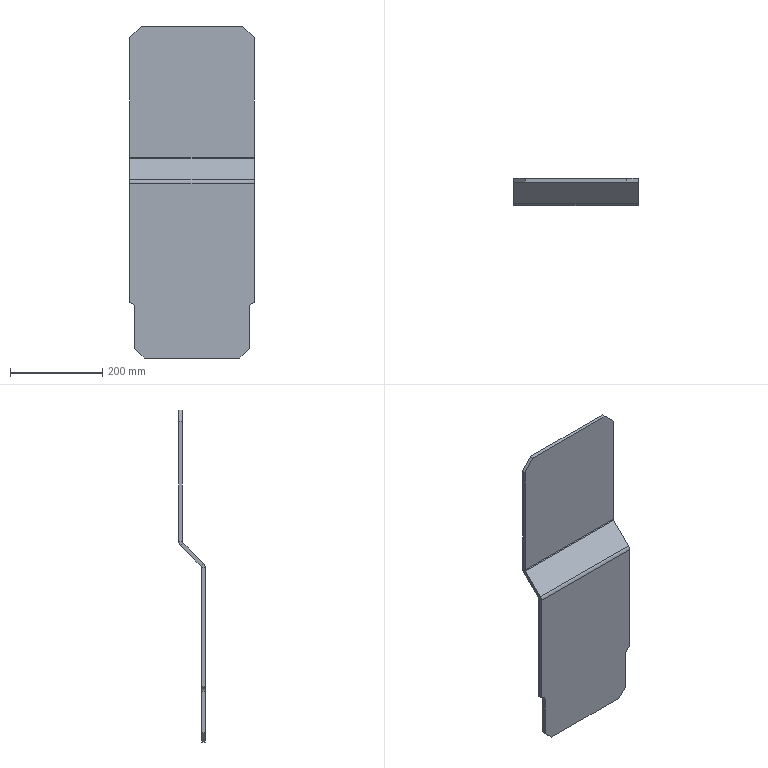Component | SolidWorks | JHK-A1001ConnectingCrossPlate-1 | 1 solid | 30 faces | box 270 x 58 x 720 mm | volume 1569543 mm3 | plane 24 | cylinder 6 | commonest cylinder face diameters 8 x2 24 x2 22 x2 | material Q235A
STEP:
#1=COLOUR_RGB('',0.7922,0.8196,0.9333);
#2=FILL_AREA_STYLE_COLOUR('',#1);
#3=FILL_AREA_STYLE('',(#2));
#4=SURFACE_STYLE_FILL_AREA(#3);
#5=SURFACE_SIDE_STYLE('',(#4));
#6=SURFACE_STYLE_USAGE(.BOTH.,#5);
#7=PRESENTATION_STYLE_ASSIGNMENT((#6));
#8=CARTESIAN_POINT('',(5.315,6.279,2.421));
#9=VERTEX_POINT('',#8);
#10=CARTESIAN_POINT('',(5.315,6.056,2.643));
#11=VERTEX_POINT('',#10);
#12=CARTESIAN_POINT('',(5.315,6.279,2.421));
#13=DIRECTION('',(0.,-0.7071,0.7071));
#14=VECTOR('',#13,39.37);
#15=LINE('',#12,#14);
#16=EDGE_CURVE('',#9,#11,#15,.T.);
#17=ORIENTED_EDGE('',*,*,#16,.F.);
#18=CARTESIAN_POINT('',(5.315,6.417,2.755));
#19=VERTEX_POINT('',#18);
#20=CARTESIAN_POINT('',(5.315,5.945,2.755));
#21=DIRECTION('',(-1.,0.,0.));
#22=DIRECTION('',(0.,0.,-1.));
#23=AXIS2_PLACEMENT_3D('',#20,#21,#22);
#24=CIRCLE('',#23,0.4724);
#25=EDGE_CURVE('',#19,#9,#24,.T.);
#26=ORIENTED_EDGE('',*,*,#25,.F.);
#27=CARTESIAN_POINT('',(5.315,6.102,2.755));
#28=VERTEX_POINT('',#27);
#29=CARTESIAN_POINT('',(5.315,6.102,2.755));
#30=DIRECTION('',(0.,1.,0.));
#31=VECTOR('',#30,39.37);
#32=LINE('',#29,#31);
#33=EDGE_CURVE('',#28,#19,#32,.T.);
#34=ORIENTED_EDGE('',*,*,#33,.F.);
#35=CARTESIAN_POINT('',(5.315,5.945,2.755));
#36=DIRECTION('',(-1.,0.,0.));
#37=DIRECTION('',(0.,0.,-1.));
#38=AXIS2_PLACEMENT_3D('',#35,#36,#37);
#39=CIRCLE('',#38,0.1575);
#40=EDGE_CURVE('',#28,#11,#39,.T.);
#41=ORIENTED_EDGE('',*,*,#40,.T.);
#42=EDGE_LOOP('',(#17,#26,#34,#41));
#43=FACE_OUTER_BOUND('',#42,.T.);
#44=CARTESIAN_POINT('',(5.315,6.279,2.421));
#45=DIRECTION('',(1.,0.,0.));
#46=DIRECTION('',(0.,0.,-1.));
#47=AXIS2_PLACEMENT_3D('',#44,#45,#46);
#48=PLANE('',#47);
#49=ADVANCED_FACE('',(#43),#48,.T.);
#50=CARTESIAN_POINT('',(5.315,4.495,0.6367));
#51=VERTEX_POINT('',#50);
#52=CARTESIAN_POINT('',(5.315,6.417,2.559));
#53=DIRECTION('',(0.,-0.7071,-0.7071));
#54=VECTOR('',#53,39.37);
#55=LINE('',#52,#54);
#56=EDGE_CURVE('',#9,#51,#55,.T.);
#57=ORIENTED_EDGE('',*,*,#56,.F.);
#58=ORIENTED_EDGE('',*,*,#16,.T.);
#59=CARTESIAN_POINT('',(5.315,4.272,0.8594));
#60=VERTEX_POINT('',#59);
#61=CARTESIAN_POINT('',(5.315,6.195,2.782));
#62=DIRECTION('',(0.,-0.7071,-0.7071));
#63=VECTOR('',#62,39.37);
#64=LINE('',#61,#63);
#65=EDGE_CURVE('',#11,#60,#64,.T.);
#66=ORIENTED_EDGE('',*,*,#65,.T.);
#67=CARTESIAN_POINT('',(5.315,4.272,0.8594));
#68=DIRECTION('',(0.,0.7071,-0.7071));
#69=VECTOR('',#68,39.37);
#70=LINE('',#67,#69);
#71=EDGE_CURVE('',#60,#51,#70,.T.);
#72=ORIENTED_EDGE('',*,*,#71,.T.);
#73=EDGE_LOOP('',(#57,#58,#66,#72));
#74=FACE_OUTER_BOUND('',#73,.T.);
#75=CARTESIAN_POINT('',(5.315,6.102,2.755));
#76=DIRECTION('',(1.,0.,0.));
#77=DIRECTION('',(0.,0.,-1.));
#78=AXIS2_PLACEMENT_3D('',#75,#76,#77);
#79=PLANE('',#78);
#80=ADVANCED_FACE('',(#74),#79,.T.);
#81=CARTESIAN_POINT('',(-5.315,6.417,2.755));
#82=VERTEX_POINT('',#81);
#83=CARTESIAN_POINT('',(-5.315,6.102,2.755));
#84=VERTEX_POINT('',#83);
#85=CARTESIAN_POINT('',(-5.315,6.417,2.755));
#86=DIRECTION('',(0.,-1.,-0.));
#87=VECTOR('',#86,39.37);
#88=LINE('',#85,#87);
#89=EDGE_CURVE('',#82,#84,#88,.T.);
#90=ORIENTED_EDGE('',*,*,#89,.F.);
#91=CARTESIAN_POINT('',(-5.315,6.279,2.421));
#92=VERTEX_POINT('',#91);
#93=CARTESIAN_POINT('',(-5.315,5.945,2.755));
#94=DIRECTION('',(-1.,0.,0.));
#95=DIRECTION('',(0.,0.,-1.));
#96=AXIS2_PLACEMENT_3D('',#93,#94,#95);
#97=CIRCLE('',#96,0.4724);
#98=EDGE_CURVE('',#82,#92,#97,.T.);
#99=ORIENTED_EDGE('',*,*,#98,.T.);
#100=CARTESIAN_POINT('',(-5.315,6.056,2.643));
#101=VERTEX_POINT('',#100);
#102=CARTESIAN_POINT('',(-5.315,6.056,2.643));
#103=DIRECTION('',(0.,0.7071,-0.7071));
#104=VECTOR('',#103,39.37);
#105=LINE('',#102,#104);
#106=EDGE_CURVE('',#101,#92,#105,.T.);
#107=ORIENTED_EDGE('',*,*,#106,.F.);
#108=CARTESIAN_POINT('',(-5.315,5.945,2.755));
#109=DIRECTION('',(-1.,0.,0.));
#110=DIRECTION('',(0.,0.,-1.));
#111=AXIS2_PLACEMENT_3D('',#108,#109,#110);
#112=CIRCLE('',#111,0.1575);
#113=EDGE_CURVE('',#84,#101,#112,.T.);
#114=ORIENTED_EDGE('',*,*,#113,.F.);
#115=EDGE_LOOP('',(#90,#99,#107,#114));
#116=FACE_OUTER_BOUND('',#115,.T.);
#117=CARTESIAN_POINT('',(-5.315,6.417,2.755));
#118=DIRECTION('',(-1.,0.,0.));
#119=DIRECTION('',(0.,0.,1.));
#120=AXIS2_PLACEMENT_3D('',#117,#118,#119);
#121=PLANE('',#120);
#122=ADVANCED_FACE('',(#116),#121,.T.);
#123=CARTESIAN_POINT('',(-5.315,6.102,12.992));
#124=VERTEX_POINT('',#123);
#125=CARTESIAN_POINT('',(-5.315,6.102,13.976));
#126=DIRECTION('',(0.,0.,-1.));
#127=VECTOR('',#126,39.37);
#128=LINE('',#125,#127);
#129=EDGE_CURVE('',#124,#84,#128,.T.);
#130=ORIENTED_EDGE('',*,*,#129,.F.);
#131=CARTESIAN_POINT('',(-5.315,6.417,12.992));
#132=VERTEX_POINT('',#131);
#133=CARTESIAN_POINT('',(-5.315,6.056,12.992));
#134=DIRECTION('',(0.,1.,0.));
#135=VECTOR('',#134,39.37);
#136=LINE('',#133,#135);
#137=EDGE_CURVE('',#124,#132,#136,.T.);
#138=ORIENTED_EDGE('',*,*,#137,.T.);
#139=CARTESIAN_POINT('',(-5.315,6.417,13.976));
#140=DIRECTION('',(0.,0.,-1.));
#141=VECTOR('',#140,39.37);
#142=LINE('',#139,#141);
#143=EDGE_CURVE('',#132,#82,#142,.T.);
#144=ORIENTED_EDGE('',*,*,#143,.T.);
#145=ORIENTED_EDGE('',*,*,#89,.T.);
#146=EDGE_LOOP('',(#130,#138,#144,#145));
#147=FACE_OUTER_BOUND('',#146,.T.);
#148=CARTESIAN_POINT('',(-5.315,6.056,2.643));
#149=DIRECTION('',(-1.,0.,0.));
#150=DIRECTION('',(0.,0.,1.));
#151=AXIS2_PLACEMENT_3D('',#148,#149,#150);
#152=PLANE('',#151);
#153=ADVANCED_FACE('',(#147),#152,.T.);
#154=CARTESIAN_POINT('',(5.315,4.449,0.5253));
#155=VERTEX_POINT('',#154);
#156=CARTESIAN_POINT('',(5.315,4.134,0.5253));
#157=VERTEX_POINT('',#156);
#158=CARTESIAN_POINT('',(5.315,4.449,0.5253));
#159=DIRECTION('',(0.,-1.,0.));
#160=VECTOR('',#159,39.37);
#161=LINE('',#158,#160);
#162=EDGE_CURVE('',#155,#157,#161,.T.);
#163=ORIENTED_EDGE('',*,*,#162,.F.);
#164=CARTESIAN_POINT('',(5.315,4.606,0.5253));
#165=DIRECTION('',(1.,0.,0.));
#166=DIRECTION('',(0.,0.,1.));
#167=AXIS2_PLACEMENT_3D('',#164,#165,#166);
#168=CIRCLE('',#167,0.1575);
#169=EDGE_CURVE('',#51,#155,#168,.T.);
#170=ORIENTED_EDGE('',*,*,#169,.F.);
#171=ORIENTED_EDGE('',*,*,#71,.F.);
#172=CARTESIAN_POINT('',(5.315,4.606,0.5253));
#173=DIRECTION('',(1.,0.,0.));
#174=DIRECTION('',(0.,0.,-1.));
#175=AXIS2_PLACEMENT_3D('',#172,#173,#174);
#176=CIRCLE('',#175,0.4724);
#177=EDGE_CURVE('',#60,#157,#176,.T.);
#178=ORIENTED_EDGE('',*,*,#177,.T.);
#179=EDGE_LOOP('',(#163,#170,#171,#178));
#180=FACE_OUTER_BOUND('',#179,.T.);
#181=CARTESIAN_POINT('',(5.315,4.449,0.5253));
#182=DIRECTION('',(1.,0.,0.));
#183=DIRECTION('',(0.,0.,-1.));
#184=AXIS2_PLACEMENT_3D('',#181,#182,#183);
#185=PLANE('',#184);
#186=ADVANCED_FACE('',(#180),#185,.T.);
#187=CARTESIAN_POINT('',(5.315,4.134,-9.646));
#188=VERTEX_POINT('',#187);
#189=CARTESIAN_POINT('',(5.315,4.449,-9.646));
#190=VERTEX_POINT('',#189);
#191=CARTESIAN_POINT('',(5.315,4.134,-9.646));
#192=DIRECTION('',(0.,1.,0.));
#193=VECTOR('',#192,39.37);
#194=LINE('',#191,#193);
#195=EDGE_CURVE('',#188,#190,#194,.T.);
#196=ORIENTED_EDGE('',*,*,#195,.T.);
#197=CARTESIAN_POINT('',(5.315,4.449,0.5906));
#198=DIRECTION('',(0.,0.,-1.));
#199=VECTOR('',#198,39.37);
#200=LINE('',#197,#199);
#201=EDGE_CURVE('',#155,#190,#200,.T.);
#202=ORIENTED_EDGE('',*,*,#201,.F.);
#203=ORIENTED_EDGE('',*,*,#162,.T.);
#204=CARTESIAN_POINT('',(5.315,4.134,0.5906));
#205=DIRECTION('',(0.,0.,-1.));
#206=VECTOR('',#205,39.37);
#207=LINE('',#204,#206);
#208=EDGE_CURVE('',#157,#188,#207,.T.);
#209=ORIENTED_EDGE('',*,*,#208,.T.);
#210=EDGE_LOOP('',(#196,#202,#203,#209));
#211=FACE_OUTER_BOUND('',#210,.T.);
#212=CARTESIAN_POINT('',(5.315,4.272,0.8594));
#213=DIRECTION('',(1.,0.,0.));
#214=DIRECTION('',(0.,0.,-1.));
#215=AXIS2_PLACEMENT_3D('',#212,#213,#214);
#216=PLANE('',#215);
#217=ADVANCED_FACE('',(#211),#216,.T.);
#218=CARTESIAN_POINT('',(-5.315,4.495,0.6367));
#219=VERTEX_POINT('',#218);
#220=CARTESIAN_POINT('',(-5.315,4.272,0.8594));
#221=VERTEX_POINT('',#220);
#222=CARTESIAN_POINT('',(-5.315,4.495,0.6367));
#223=DIRECTION('',(0.,-0.7071,0.7071));
#224=VECTOR('',#223,39.37);
#225=LINE('',#222,#224);
#226=EDGE_CURVE('',#219,#221,#225,.T.);
#227=ORIENTED_EDGE('',*,*,#226,.F.);
#228=CARTESIAN_POINT('',(-5.315,4.449,0.5253));
#229=VERTEX_POINT('',#228);
#230=CARTESIAN_POINT('',(-5.315,4.606,0.5253));
#231=DIRECTION('',(1.,0.,0.));
#232=DIRECTION('',(0.,0.,1.));
#233=AXIS2_PLACEMENT_3D('',#230,#231,#232);
#234=CIRCLE('',#233,0.1575);
#235=EDGE_CURVE('',#219,#229,#234,.T.);
#236=ORIENTED_EDGE('',*,*,#235,.T.);
#237=CARTESIAN_POINT('',(-5.315,4.134,0.5253));
#238=VERTEX_POINT('',#237);
#239=CARTESIAN_POINT('',(-5.315,4.134,0.5253));
#240=DIRECTION('',(0.,1.,0.));
#241=VECTOR('',#240,39.37);
#242=LINE('',#239,#241);
#243=EDGE_CURVE('',#238,#229,#242,.T.);
#244=ORIENTED_EDGE('',*,*,#243,.F.);
#245=CARTESIAN_POINT('',(-5.315,4.606,0.5253));
#246=DIRECTION('',(1.,0.,0.));
#247=DIRECTION('',(0.,0.,-1.));
#248=AXIS2_PLACEMENT_3D('',#245,#246,#247);
#249=CIRCLE('',#248,0.4724);
#250=EDGE_CURVE('',#221,#238,#249,.T.);
#251=ORIENTED_EDGE('',*,*,#250,.F.);
#252=EDGE_LOOP('',(#227,#236,#244,#251));
#253=FACE_OUTER_BOUND('',#252,.T.);
#254=CARTESIAN_POINT('',(-5.315,4.495,0.6367));
#255=DIRECTION('',(-1.,0.,0.));
#256=DIRECTION('',(0.,0.,1.));
#257=AXIS2_PLACEMENT_3D('',#254,#255,#256);
#258=PLANE('',#257);
#259=ADVANCED_FACE('',(#253),#258,.T.);
#260=CARTESIAN_POINT('',(-5.315,6.417,2.559));
#261=DIRECTION('',(0.,-0.7071,-0.7071));
#262=VECTOR('',#261,39.37);
#263=LINE('',#260,#262);
#264=EDGE_CURVE('',#92,#219,#263,.T.);
#265=ORIENTED_EDGE('',*,*,#264,.T.);
#266=ORIENTED_EDGE('',*,*,#226,.T.);
#267=CARTESIAN_POINT('',(-5.315,6.195,2.782));
#268=DIRECTION('',(0.,-0.7071,-0.7071));
#269=VECTOR('',#268,39.37);
#270=LINE('',#267,#269);
#271=EDGE_CURVE('',#101,#221,#270,.T.);
#272=ORIENTED_EDGE('',*,*,#271,.F.);
#273=ORIENTED_EDGE('',*,*,#106,.T.);
#274=EDGE_LOOP('',(#265,#266,#272,#273));
#275=FACE_OUTER_BOUND('',#274,.T.);
#276=CARTESIAN_POINT('',(-5.315,4.134,0.5253));
#277=DIRECTION('',(-1.,0.,0.));
#278=DIRECTION('',(0.,0.,1.));
#279=AXIS2_PLACEMENT_3D('',#276,#277,#278);
#280=PLANE('',#279);
#281=ADVANCED_FACE('',(#275),#280,.T.);
#282=CARTESIAN_POINT('',(-4.882,4.134,-10.079));
#283=VERTEX_POINT('',#282);
#284=CARTESIAN_POINT('',(-4.882,4.134,-13.583));
#285=VERTEX_POINT('',#284);
#286=CARTESIAN_POINT('',(-4.882,4.134,-14.37));
#287=DIRECTION('',(-0.,0.,-1.));
#288=VECTOR('',#287,39.37);
#289=LINE('',#286,#288);
#290=EDGE_CURVE('',#283,#285,#289,.T.);
#291=ORIENTED_EDGE('',*,*,#290,.T.);
#292=CARTESIAN_POINT('',(-4.094,4.134,-14.37));
#293=VERTEX_POINT('',#292);
#294=CARTESIAN_POINT('',(-4.094,4.134,-14.37));
#295=DIRECTION('',(0.7071,0.,-0.7071));
#296=VECTOR('',#295,39.37);
#297=LINE('',#294,#296);
#298=EDGE_CURVE('',#285,#293,#297,.T.);
#299=ORIENTED_EDGE('',*,*,#298,.T.);
#300=CARTESIAN_POINT('',(4.094,4.134,-14.37));
#301=VERTEX_POINT('',#300);
#302=CARTESIAN_POINT('',(5.315,4.134,-14.37));
#303=DIRECTION('',(-1.,0.,0.));
#304=VECTOR('',#303,39.37);
#305=LINE('',#302,#304);
#306=EDGE_CURVE('',#301,#293,#305,.T.);
#307=ORIENTED_EDGE('',*,*,#306,.F.);
#308=CARTESIAN_POINT('',(4.882,4.134,-13.583));
#309=VERTEX_POINT('',#308);
#310=CARTESIAN_POINT('',(4.882,4.134,-13.583));
#311=DIRECTION('',(0.7071,-0.,0.7071));
#312=VECTOR('',#311,39.37);
#313=LINE('',#310,#312);
#314=EDGE_CURVE('',#301,#309,#313,.T.);
#315=ORIENTED_EDGE('',*,*,#314,.T.);
#316=CARTESIAN_POINT('',(4.882,4.134,-10.079));
#317=VERTEX_POINT('',#316);
#318=CARTESIAN_POINT('',(4.882,4.134,-14.37));
#319=DIRECTION('',(0.,0.,1.));
#320=VECTOR('',#319,39.37);
#321=LINE('',#318,#320);
#322=EDGE_CURVE('',#309,#317,#321,.T.);
#323=ORIENTED_EDGE('',*,*,#322,.T.);
#324=CARTESIAN_POINT('',(5.315,4.134,-10.079));
#325=DIRECTION('',(0.,1.,0.));
#326=DIRECTION('',(0.,0.,1.));
#327=AXIS2_PLACEMENT_3D('',#324,#325,#326);
#328=CIRCLE('',#327,0.4331);
#329=EDGE_CURVE('',#317,#188,#328,.T.);
#330=ORIENTED_EDGE('',*,*,#329,.T.);
#331=ORIENTED_EDGE('',*,*,#208,.F.);
#332=CARTESIAN_POINT('',(5.315,4.134,0.5253));
#333=DIRECTION('',(-1.,0.,0.));
#334=VECTOR('',#333,39.37);
#335=LINE('',#332,#334);
#336=EDGE_CURVE('',#157,#238,#335,.T.);
#337=ORIENTED_EDGE('',*,*,#336,.T.);
#338=CARTESIAN_POINT('',(-5.315,4.134,-9.646));
#339=VERTEX_POINT('',#338);
#340=CARTESIAN_POINT('',(-5.315,4.134,0.5906));
#341=DIRECTION('',(0.,0.,-1.));
#342=VECTOR('',#341,39.37);
#343=LINE('',#340,#342);
#344=EDGE_CURVE('',#238,#339,#343,.T.);
#345=ORIENTED_EDGE('',*,*,#344,.T.);
#346=CARTESIAN_POINT('',(-5.315,4.134,-10.079));
#347=DIRECTION('',(0.,1.,0.));
#348=DIRECTION('',(0.,0.,1.));
#349=AXIS2_PLACEMENT_3D('',#346,#347,#348);
#350=CIRCLE('',#349,0.4331);
#351=EDGE_CURVE('',#339,#283,#350,.T.);
#352=ORIENTED_EDGE('',*,*,#351,.T.);
#353=EDGE_LOOP('',(#291,#299,#307,#315,#323,#330,#331,#337,#345,#352));
#354=FACE_OUTER_BOUND('',#353,.T.);
#355=CARTESIAN_POINT('',(5.315,4.134,0.5906));
#356=DIRECTION('',(0.,1.,0.));
#357=DIRECTION('',(0.,-0.,1.));
#358=AXIS2_PLACEMENT_3D('',#355,#356,#357);
#359=PLANE('',#358);
#360=ADVANCED_FACE('',(#354),#359,.F.);
#361=ORIENTED_EDGE('',*,*,#306,.T.);
#362=CARTESIAN_POINT('',(-4.094,4.449,-14.37));
#363=VERTEX_POINT('',#362);
#364=CARTESIAN_POINT('',(-4.094,4.449,-14.37));
#365=DIRECTION('',(0.,1.,0.));
#366=VECTOR('',#365,39.37);
#367=LINE('',#364,#366);
#368=EDGE_CURVE('',#293,#363,#367,.T.);
#369=ORIENTED_EDGE('',*,*,#368,.T.);
#370=CARTESIAN_POINT('',(4.094,4.449,-14.37));
#371=VERTEX_POINT('',#370);
#372=CARTESIAN_POINT('',(5.315,4.449,-14.37));
#373=DIRECTION('',(-1.,0.,0.));
#374=VECTOR('',#373,39.37);
#375=LINE('',#372,#374);
#376=EDGE_CURVE('',#371,#363,#375,.T.);
#377=ORIENTED_EDGE('',*,*,#376,.F.);
#378=CARTESIAN_POINT('',(4.094,4.134,-14.37));
#379=DIRECTION('',(0.,-1.,0.));
#380=VECTOR('',#379,39.37);
#381=LINE('',#378,#380);
#382=EDGE_CURVE('',#371,#301,#381,.T.);
#383=ORIENTED_EDGE('',*,*,#382,.T.);
#384=EDGE_LOOP('',(#361,#369,#377,#383));
#385=FACE_OUTER_BOUND('',#384,.T.);
#386=CARTESIAN_POINT('',(5.315,4.449,-14.37));
#387=DIRECTION('',(0.,0.,-1.));
#388=DIRECTION('',(-1.,0.,0.));
#389=AXIS2_PLACEMENT_3D('',#386,#387,#388);
#390=PLANE('',#389);
#391=ADVANCED_FACE('',(#385),#390,.T.);
#392=ORIENTED_EDGE('',*,*,#376,.T.);
#393=CARTESIAN_POINT('',(-4.882,4.449,-13.583));
#394=VERTEX_POINT('',#393);
#395=CARTESIAN_POINT('',(-6.87,4.449,-11.594));
#396=DIRECTION('',(-0.7071,-0.,0.7071));
#397=VECTOR('',#396,39.37);
#398=LINE('',#395,#397);
#399=EDGE_CURVE('',#363,#394,#398,.T.);
#400=ORIENTED_EDGE('',*,*,#399,.T.);
#401=CARTESIAN_POINT('',(-4.882,4.449,-10.079));
#402=VERTEX_POINT('',#401);
#403=CARTESIAN_POINT('',(-4.882,4.449,-14.37));
#404=DIRECTION('',(-0.,0.,-1.));
#405=VECTOR('',#404,39.37);
#406=LINE('',#403,#405);
#407=EDGE_CURVE('',#402,#394,#406,.T.);
#408=ORIENTED_EDGE('',*,*,#407,.F.);
#409=CARTESIAN_POINT('',(-5.315,4.449,-9.646));
#410=VERTEX_POINT('',#409);
#411=CARTESIAN_POINT('',(-5.315,4.449,-10.079));
#412=DIRECTION('',(0.,-1.,-0.));
#413=DIRECTION('',(0.,0.,1.));
#414=AXIS2_PLACEMENT_3D('',#411,#412,#413);
#415=CIRCLE('',#414,0.4331);
#416=EDGE_CURVE('',#402,#410,#415,.T.);
#417=ORIENTED_EDGE('',*,*,#416,.T.);
#418=CARTESIAN_POINT('',(-5.315,4.449,0.5906));
#419=DIRECTION('',(0.,0.,-1.));
#420=VECTOR('',#419,39.37);
#421=LINE('',#418,#420);
#422=EDGE_CURVE('',#229,#410,#421,.T.);
#423=ORIENTED_EDGE('',*,*,#422,.F.);
#424=CARTESIAN_POINT('',(5.315,4.449,0.5253));
#425=DIRECTION('',(-1.,0.,0.));
#426=VECTOR('',#425,39.37);
#427=LINE('',#424,#426);
#428=EDGE_CURVE('',#155,#229,#427,.T.);
#429=ORIENTED_EDGE('',*,*,#428,.F.);
#430=ORIENTED_EDGE('',*,*,#201,.T.);
#431=CARTESIAN_POINT('',(4.882,4.449,-10.079));
#432=VERTEX_POINT('',#431);
#433=CARTESIAN_POINT('',(5.315,4.449,-10.079));
#434=DIRECTION('',(0.,-1.,-0.));
#435=DIRECTION('',(0.,0.,1.));
#436=AXIS2_PLACEMENT_3D('',#433,#434,#435);
#437=CIRCLE('',#436,0.4331);
#438=EDGE_CURVE('',#190,#432,#437,.T.);
#439=ORIENTED_EDGE('',*,*,#438,.T.);
#440=CARTESIAN_POINT('',(4.882,4.449,-13.583));
#441=VERTEX_POINT('',#440);
#442=CARTESIAN_POINT('',(4.882,4.449,-14.37));
#443=DIRECTION('',(0.,0.,1.));
#444=VECTOR('',#443,39.37);
#445=LINE('',#442,#444);
#446=EDGE_CURVE('',#441,#432,#445,.T.);
#447=ORIENTED_EDGE('',*,*,#446,.F.);
#448=CARTESIAN_POINT('',(12.185,4.449,-6.28));
#449=DIRECTION('',(-0.7071,0.,-0.7071));
#450=VECTOR('',#449,39.37);
#451=LINE('',#448,#450);
#452=EDGE_CURVE('',#441,#371,#451,.T.);
#453=ORIENTED_EDGE('',*,*,#452,.T.);
#454=EDGE_LOOP('',(#392,#400,#408,#417,#423,#429,#430,#439,#447,#453));
#455=FACE_OUTER_BOUND('',#454,.T.);
#456=CARTESIAN_POINT('',(5.315,4.449,0.5906));
#457=DIRECTION('',(0.,1.,0.));
#458=DIRECTION('',(0.,-0.,1.));
#459=AXIS2_PLACEMENT_3D('',#456,#457,#458);
#460=PLANE('',#459);
#461=ADVANCED_FACE('',(#455),#460,.T.);
#462=ORIENTED_EDGE('',*,*,#235,.F.);
#463=CARTESIAN_POINT('',(5.315,4.495,0.6367));
#464=DIRECTION('',(-1.,0.,0.));
#465=VECTOR('',#464,39.37);
#466=LINE('',#463,#465);
#467=EDGE_CURVE('',#51,#219,#466,.T.);
#468=ORIENTED_EDGE('',*,*,#467,.F.);
#469=ORIENTED_EDGE('',*,*,#169,.T.);
#470=ORIENTED_EDGE('',*,*,#428,.T.);
#471=EDGE_LOOP('',(#462,#468,#469,#470));
#472=FACE_OUTER_BOUND('',#471,.T.);
#473=CARTESIAN_POINT('',(5.315,4.606,0.5253));
#474=DIRECTION('',(-1.,0.,0.));
#475=DIRECTION('',(0.,0.,1.));
#476=AXIS2_PLACEMENT_3D('',#473,#474,#475);
#477=CYLINDRICAL_SURFACE('',#476,0.1575);
#478=ADVANCED_FACE('',(#472),#477,.F.);
#479=ORIENTED_EDGE('',*,*,#264,.F.);
#480=CARTESIAN_POINT('',(5.315,6.279,2.421));
#481=DIRECTION('',(-1.,0.,0.));
#482=VECTOR('',#481,39.37);
#483=LINE('',#480,#482);
#484=EDGE_CURVE('',#9,#92,#483,.T.);
#485=ORIENTED_EDGE('',*,*,#484,.F.);
#486=ORIENTED_EDGE('',*,*,#56,.T.);
#487=ORIENTED_EDGE('',*,*,#467,.T.);
#488=EDGE_LOOP('',(#479,#485,#486,#487));
#489=FACE_OUTER_BOUND('',#488,.T.);
#490=CARTESIAN_POINT('',(5.315,6.417,2.559));
#491=DIRECTION('',(0.,0.7071,-0.7071));
#492=DIRECTION('',(0.,0.7071,0.7071));
#493=AXIS2_PLACEMENT_3D('',#490,#491,#492);
#494=PLANE('',#493);
#495=ADVANCED_FACE('',(#489),#494,.T.);
#496=ORIENTED_EDGE('',*,*,#98,.F.);
#497=CARTESIAN_POINT('',(5.315,6.417,2.755));
#498=DIRECTION('',(-1.,0.,0.));
#499=VECTOR('',#498,39.37);
#500=LINE('',#497,#499);
#501=EDGE_CURVE('',#19,#82,#500,.T.);
#502=ORIENTED_EDGE('',*,*,#501,.F.);
#503=ORIENTED_EDGE('',*,*,#25,.T.);
#504=ORIENTED_EDGE('',*,*,#484,.T.);
#505=EDGE_LOOP('',(#496,#502,#503,#504));
#506=FACE_OUTER_BOUND('',#505,.T.);
#507=CARTESIAN_POINT('',(5.315,5.945,2.755));
#508=DIRECTION('',(-1.,0.,0.));
#509=DIRECTION('',(0.,0.,1.));
#510=AXIS2_PLACEMENT_3D('',#507,#508,#509);
#511=CYLINDRICAL_SURFACE('',#510,0.4724);
#512=ADVANCED_FACE('',(#506),#511,.T.);
#513=ORIENTED_EDGE('',*,*,#143,.F.);
#514=CARTESIAN_POINT('',(-4.331,6.417,13.976));
#515=VERTEX_POINT('',#514);
#516=CARTESIAN_POINT('',(0.4921,6.417,18.799));
#517=DIRECTION('',(0.7071,0.,0.7071));
#518=VECTOR('',#517,39.37);
#519=LINE('',#516,#518);
#520=EDGE_CURVE('',#132,#515,#519,.T.);
#521=ORIENTED_EDGE('',*,*,#520,.T.);
#522=CARTESIAN_POINT('',(4.331,6.417,13.976));
#523=VERTEX_POINT('',#522);
#524=CARTESIAN_POINT('',(5.315,6.417,13.976));
#525=DIRECTION('',(-1.,0.,0.));
#526=VECTOR('',#525,39.37);
#527=LINE('',#524,#526);
#528=EDGE_CURVE('',#523,#515,#527,.T.);
#529=ORIENTED_EDGE('',*,*,#528,.F.);
#530=CARTESIAN_POINT('',(5.315,6.417,12.992));
#531=VERTEX_POINT('',#530);
#532=CARTESIAN_POINT('',(4.823,6.417,13.484));
#533=DIRECTION('',(0.7071,0.,-0.7071));
#534=VECTOR('',#533,39.37);
#535=LINE('',#532,#534);
#536=EDGE_CURVE('',#523,#531,#535,.T.);
#537=ORIENTED_EDGE('',*,*,#536,.T.);
#538=CARTESIAN_POINT('',(5.315,6.417,13.976));
#539=DIRECTION('',(0.,0.,-1.));
#540=VECTOR('',#539,39.37);
#541=LINE('',#538,#540);
#542=EDGE_CURVE('',#531,#19,#541,.T.);
#543=ORIENTED_EDGE('',*,*,#542,.T.);
#544=ORIENTED_EDGE('',*,*,#501,.T.);
#545=EDGE_LOOP('',(#513,#521,#529,#537,#543,#544));
#546=FACE_OUTER_BOUND('',#545,.T.);
#547=CARTESIAN_POINT('',(5.315,6.417,13.976));
#548=DIRECTION('',(0.,1.,0.));
#549=DIRECTION('',(0.,0.,1.));
#550=AXIS2_PLACEMENT_3D('',#547,#548,#549);
#551=PLANE('',#550);
#552=ADVANCED_FACE('',(#546),#551,.T.);
#553=ORIENTED_EDGE('',*,*,#528,.T.);
#554=CARTESIAN_POINT('',(-4.331,6.102,13.976));
#555=VERTEX_POINT('',#554);
#556=CARTESIAN_POINT('',(-4.331,6.102,13.976));
#557=DIRECTION('',(0.,-1.,0.));
#558=VECTOR('',#557,39.37);
#559=LINE('',#556,#558);
#560=EDGE_CURVE('',#515,#555,#559,.T.);
#561=ORIENTED_EDGE('',*,*,#560,.T.);
#562=CARTESIAN_POINT('',(4.331,6.102,13.976));
#563=VERTEX_POINT('',#562);
#564=CARTESIAN_POINT('',(5.315,6.102,13.976));
#565=DIRECTION('',(-1.,0.,0.));
#566=VECTOR('',#565,39.37);
#567=LINE('',#564,#566);
#568=EDGE_CURVE('',#563,#555,#567,.T.);
#569=ORIENTED_EDGE('',*,*,#568,.F.);
#570=CARTESIAN_POINT('',(4.331,6.417,13.976));
#571=DIRECTION('',(0.,1.,0.));
#572=VECTOR('',#571,39.37);
#573=LINE('',#570,#572);
#574=EDGE_CURVE('',#563,#523,#573,.T.);
#575=ORIENTED_EDGE('',*,*,#574,.T.);
#576=EDGE_LOOP('',(#553,#561,#569,#575));
#577=FACE_OUTER_BOUND('',#576,.T.);
#578=CARTESIAN_POINT('',(5.315,6.102,13.976));
#579=DIRECTION('',(0.,0.,1.));
#580=DIRECTION('',(1.,0.,0.));
#581=AXIS2_PLACEMENT_3D('',#578,#579,#580);
#582=PLANE('',#581);
#583=ADVANCED_FACE('',(#577),#582,.T.);
#584=ORIENTED_EDGE('',*,*,#568,.T.);
#585=CARTESIAN_POINT('',(-5.315,6.102,12.992));
#586=DIRECTION('',(-0.7071,0.,-0.7071));
#587=VECTOR('',#586,39.37);
#588=LINE('',#585,#587);
#589=EDGE_CURVE('',#555,#124,#588,.T.);
#590=ORIENTED_EDGE('',*,*,#589,.T.);
#591=ORIENTED_EDGE('',*,*,#129,.T.);
#592=CARTESIAN_POINT('',(5.315,6.102,2.755));
#593=DIRECTION('',(-1.,0.,0.));
#594=VECTOR('',#593,39.37);
#595=LINE('',#592,#594);
#596=EDGE_CURVE('',#28,#84,#595,.T.);
#597=ORIENTED_EDGE('',*,*,#596,.F.);
#598=CARTESIAN_POINT('',(5.315,6.102,12.992));
#599=VERTEX_POINT('',#598);
#600=CARTESIAN_POINT('',(5.315,6.102,13.976));
#601=DIRECTION('',(0.,0.,-1.));
#602=VECTOR('',#601,39.37);
#603=LINE('',#600,#602);
#604=EDGE_CURVE('',#599,#28,#603,.T.);
#605=ORIENTED_EDGE('',*,*,#604,.F.);
#606=CARTESIAN_POINT('',(4.331,6.102,13.976));
#607=DIRECTION('',(-0.7071,0.,0.7071));
#608=VECTOR('',#607,39.37);
#609=LINE('',#606,#608);
#610=EDGE_CURVE('',#599,#563,#609,.T.);
#611=ORIENTED_EDGE('',*,*,#610,.T.);
#612=EDGE_LOOP('',(#584,#590,#591,#597,#605,#611));
#613=FACE_OUTER_BOUND('',#612,.T.);
#614=CARTESIAN_POINT('',(5.315,6.102,13.976));
#615=DIRECTION('',(0.,1.,0.));
#616=DIRECTION('',(0.,0.,1.));
#617=AXIS2_PLACEMENT_3D('',#614,#615,#616);
#618=PLANE('',#617);
#619=ADVANCED_FACE('',(#613),#618,.F.);
#620=ORIENTED_EDGE('',*,*,#113,.T.);
#621=CARTESIAN_POINT('',(5.315,6.056,2.643));
#622=DIRECTION('',(-1.,0.,0.));
#623=VECTOR('',#622,39.37);
#624=LINE('',#621,#623);
#625=EDGE_CURVE('',#11,#101,#624,.T.);
#626=ORIENTED_EDGE('',*,*,#625,.F.);
#627=ORIENTED_EDGE('',*,*,#40,.F.);
#628=ORIENTED_EDGE('',*,*,#596,.T.);
#629=EDGE_LOOP('',(#620,#626,#627,#628));
#630=FACE_OUTER_BOUND('',#629,.T.);
#631=CARTESIAN_POINT('',(5.315,5.945,2.755));
#632=DIRECTION('',(-1.,0.,0.));
#633=DIRECTION('',(0.,0.,1.));
#634=AXIS2_PLACEMENT_3D('',#631,#632,#633);
#635=CYLINDRICAL_SURFACE('',#634,0.1575);
#636=ADVANCED_FACE('',(#630),#635,.F.);
#637=ORIENTED_EDGE('',*,*,#271,.T.);
#638=CARTESIAN_POINT('',(5.315,4.272,0.8594));
#639=DIRECTION('',(-1.,0.,0.));
#640=VECTOR('',#639,39.37);
#641=LINE('',#638,#640);
#642=EDGE_CURVE('',#60,#221,#641,.T.);
#643=ORIENTED_EDGE('',*,*,#642,.F.);
#644=ORIENTED_EDGE('',*,*,#65,.F.);
#645=ORIENTED_EDGE('',*,*,#625,.T.);
#646=EDGE_LOOP('',(#637,#643,#644,#645));
#647=FACE_OUTER_BOUND('',#646,.T.);
#648=CARTESIAN_POINT('',(5.315,6.195,2.782));
#649=DIRECTION('',(0.,0.7071,-0.7071));
#650=DIRECTION('',(0.,0.7071,0.7071));
#651=AXIS2_PLACEMENT_3D('',#648,#649,#650);
#652=PLANE('',#651);
#653=ADVANCED_FACE('',(#647),#652,.F.);
#654=ORIENTED_EDGE('',*,*,#250,.T.);
#655=ORIENTED_EDGE('',*,*,#336,.F.);
#656=ORIENTED_EDGE('',*,*,#177,.F.);
#657=ORIENTED_EDGE('',*,*,#642,.T.);
#658=EDGE_LOOP('',(#654,#655,#656,#657));
#659=FACE_OUTER_BOUND('',#658,.T.);
#660=CARTESIAN_POINT('',(5.315,4.606,0.5253));
#661=DIRECTION('',(-1.,0.,0.));
#662=DIRECTION('',(0.,0.,1.));
#663=AXIS2_PLACEMENT_3D('',#660,#661,#662);
#664=CYLINDRICAL_SURFACE('',#663,0.4724);
#665=ADVANCED_FACE('',(#659),#664,.T.);
#666=ORIENTED_EDGE('',*,*,#542,.F.);
#667=CARTESIAN_POINT('',(5.315,6.102,12.992));
#668=DIRECTION('',(0.,-1.,0.));
#669=VECTOR('',#668,39.37);
#670=LINE('',#667,#669);
#671=EDGE_CURVE('',#531,#599,#670,.T.);
#672=ORIENTED_EDGE('',*,*,#671,.T.);
#673=ORIENTED_EDGE('',*,*,#604,.T.);
#674=ORIENTED_EDGE('',*,*,#33,.T.);
#675=EDGE_LOOP('',(#666,#672,#673,#674));
#676=FACE_OUTER_BOUND('',#675,.T.);
#677=CARTESIAN_POINT('',(5.315,4.606,0.5253));
#678=DIRECTION('',(-1.,0.,0.));
#679=DIRECTION('',(0.,0.,1.));
#680=AXIS2_PLACEMENT_3D('',#677,#678,#679);
#681=PLANE('',#680);
#682=ADVANCED_FACE('',(#676),#681,.F.);
#683=CARTESIAN_POINT('',(-5.315,4.134,-9.646));
#684=DIRECTION('',(0.,1.,0.));
#685=VECTOR('',#684,39.37);
#686=LINE('',#683,#685);
#687=EDGE_CURVE('',#339,#410,#686,.T.);
#688=ORIENTED_EDGE('',*,*,#687,.F.);
#689=ORIENTED_EDGE('',*,*,#344,.F.);
#690=ORIENTED_EDGE('',*,*,#243,.T.);
#691=ORIENTED_EDGE('',*,*,#422,.T.);
#692=EDGE_LOOP('',(#688,#689,#690,#691));
#693=FACE_OUTER_BOUND('',#692,.T.);
#694=CARTESIAN_POINT('',(-5.315,4.606,0.5253));
#695=DIRECTION('',(-1.,0.,0.));
#696=DIRECTION('',(0.,0.,1.));
#697=AXIS2_PLACEMENT_3D('',#694,#695,#696);
#698=PLANE('',#697);
#699=ADVANCED_FACE('',(#693),#698,.T.);
#700=ORIENTED_EDGE('',*,*,#407,.T.);
#701=CARTESIAN_POINT('',(-4.882,4.134,-13.583));
#702=DIRECTION('',(0.,-1.,0.));
#703=VECTOR('',#702,39.37);
#704=LINE('',#701,#703);
#705=EDGE_CURVE('',#394,#285,#704,.T.);
#706=ORIENTED_EDGE('',*,*,#705,.T.);
#707=ORIENTED_EDGE('',*,*,#290,.F.);
#708=CARTESIAN_POINT('',(-4.882,4.449,-10.079));
#709=DIRECTION('',(0.,1.,0.));
#710=VECTOR('',#709,39.37);
#711=LINE('',#708,#710);
#712=EDGE_CURVE('',#283,#402,#711,.T.);
#713=ORIENTED_EDGE('',*,*,#712,.T.);
#714=EDGE_LOOP('',(#700,#706,#707,#713));
#715=FACE_OUTER_BOUND('',#714,.T.);
#716=CARTESIAN_POINT('',(-4.882,4.134,-14.37));
#717=DIRECTION('',(1.,0.,-0.));
#718=DIRECTION('',(-0.,0.,-1.));
#719=AXIS2_PLACEMENT_3D('',#716,#717,#718);
#720=PLANE('',#719);
#721=ADVANCED_FACE('',(#715),#720,.F.);
#722=ORIENTED_EDGE('',*,*,#322,.F.);
#723=CARTESIAN_POINT('',(4.882,4.449,-13.583));
#724=DIRECTION('',(0.,1.,0.));
#725=VECTOR('',#724,39.37);
#726=LINE('',#723,#725);
#727=EDGE_CURVE('',#309,#441,#726,.T.);
#728=ORIENTED_EDGE('',*,*,#727,.T.);
#729=ORIENTED_EDGE('',*,*,#446,.T.);
#730=CARTESIAN_POINT('',(4.882,4.134,-10.079));
#731=DIRECTION('',(0.,-1.,0.));
#732=VECTOR('',#731,39.37);
#733=LINE('',#730,#732);
#734=EDGE_CURVE('',#432,#317,#733,.T.);
#735=ORIENTED_EDGE('',*,*,#734,.T.);
#736=EDGE_LOOP('',(#722,#728,#729,#735));
#737=FACE_OUTER_BOUND('',#736,.T.);
#738=CARTESIAN_POINT('',(4.882,4.134,-14.37));
#739=DIRECTION('',(-1.,0.,0.));
#740=DIRECTION('',(0.,0.,1.));
#741=AXIS2_PLACEMENT_3D('',#738,#739,#740);
#742=PLANE('',#741);
#743=ADVANCED_FACE('',(#737),#742,.F.);
#744=ORIENTED_EDGE('',*,*,#329,.F.);
#745=ORIENTED_EDGE('',*,*,#734,.F.);
#746=ORIENTED_EDGE('',*,*,#438,.F.);
#747=ORIENTED_EDGE('',*,*,#195,.F.);
#748=EDGE_LOOP('',(#744,#745,#746,#747));
#749=FACE_OUTER_BOUND('',#748,.T.);
#750=CARTESIAN_POINT('',(5.315,4.134,-10.079));
#751=DIRECTION('',(0.,-1.,0.));
#752=DIRECTION('',(0.,0.,-1.));
#753=AXIS2_PLACEMENT_3D('',#750,#751,#752);
#754=CYLINDRICAL_SURFACE('',#753,0.4331);
#755=ADVANCED_FACE('',(#749),#754,.F.);
#756=ORIENTED_EDGE('',*,*,#351,.F.);
#757=ORIENTED_EDGE('',*,*,#687,.T.);
#758=ORIENTED_EDGE('',*,*,#416,.F.);
#759=ORIENTED_EDGE('',*,*,#712,.F.);
#760=EDGE_LOOP('',(#756,#757,#758,#759));
#761=FACE_OUTER_BOUND('',#760,.T.);
#762=CARTESIAN_POINT('',(-5.315,4.134,-10.079));
#763=DIRECTION('',(0.,-1.,0.));
#764=DIRECTION('',(0.,0.,-1.));
#765=AXIS2_PLACEMENT_3D('',#762,#763,#764);
#766=CYLINDRICAL_SURFACE('',#765,0.4331);
#767=ADVANCED_FACE('',(#761),#766,.F.);
#768=ORIENTED_EDGE('',*,*,#298,.F.);
#769=ORIENTED_EDGE('',*,*,#705,.F.);
#770=ORIENTED_EDGE('',*,*,#399,.F.);
#771=ORIENTED_EDGE('',*,*,#368,.F.);
#772=EDGE_LOOP('',(#768,#769,#770,#771));
#773=FACE_OUTER_BOUND('',#772,.T.);
#774=CARTESIAN_POINT('',(-4.094,4.449,-14.37));
#775=DIRECTION('',(-0.7071,0.,-0.7071));
#776=DIRECTION('',(0.,-1.,0.));
#777=AXIS2_PLACEMENT_3D('',#774,#775,#776);
#778=PLANE('',#777);
#779=ADVANCED_FACE('',(#773),#778,.T.);
#780=ORIENTED_EDGE('',*,*,#314,.F.);
#781=ORIENTED_EDGE('',*,*,#382,.F.);
#782=ORIENTED_EDGE('',*,*,#452,.F.);
#783=ORIENTED_EDGE('',*,*,#727,.F.);
#784=EDGE_LOOP('',(#780,#781,#782,#783));
#785=FACE_OUTER_BOUND('',#784,.T.);
#786=CARTESIAN_POINT('',(4.882,4.134,-13.583));
#787=DIRECTION('',(0.7071,0.,-0.7071));
#788=DIRECTION('',(0.,-1.,0.));
#789=AXIS2_PLACEMENT_3D('',#786,#787,#788);
#790=PLANE('',#789);
#791=ADVANCED_FACE('',(#785),#790,.T.);
#792=ORIENTED_EDGE('',*,*,#589,.F.);
#793=ORIENTED_EDGE('',*,*,#560,.F.);
#794=ORIENTED_EDGE('',*,*,#520,.F.);
#795=ORIENTED_EDGE('',*,*,#137,.F.);
#796=EDGE_LOOP('',(#792,#793,#794,#795));
#797=FACE_OUTER_BOUND('',#796,.T.);
#798=CARTESIAN_POINT('',(-5.315,6.056,12.992));
#799=DIRECTION('',(0.7071,0.,-0.7071));
#800=DIRECTION('',(0.,1.,0.));
#801=AXIS2_PLACEMENT_3D('',#798,#799,#800);
#802=PLANE('',#801);
#803=ADVANCED_FACE('',(#797),#802,.F.);
#804=ORIENTED_EDGE('',*,*,#610,.F.);
#805=ORIENTED_EDGE('',*,*,#671,.F.);
#806=ORIENTED_EDGE('',*,*,#536,.F.);
#807=ORIENTED_EDGE('',*,*,#574,.F.);
#808=EDGE_LOOP('',(#804,#805,#806,#807));
#809=FACE_OUTER_BOUND('',#808,.T.);
#810=CARTESIAN_POINT('',(4.331,6.102,13.976));
#811=DIRECTION('',(0.7071,0.,0.7071));
#812=DIRECTION('',(0.,-1.,0.));
#813=AXIS2_PLACEMENT_3D('',#810,#811,#812);
#814=PLANE('',#813);
#815=ADVANCED_FACE('',(#809),#814,.T.);
#816=CLOSED_SHELL('',(#49,#80,#122,#153,#186,#217,#259,#281,#360,#391,#461,#478,#495,#512,#552,#583,#619,#636,#653,#665,#682,#699,#721,#743,#755,#767,#779,#791,#803,#815));
#817=MANIFOLD_SOLID_BREP('',#816);
#818=STYLED_ITEM('',(#7),#817);
#819=(LENGTH_UNIT()NAMED_UNIT(*)SI_UNIT($,.METRE.));
#820=LENGTH_MEASURE_WITH_UNIT(LENGTH_MEASURE(0.0254),#819);
#821=DIMENSIONAL_EXPONENTS(1.,0.,0.,0.,0.,0.,0.);
#822=(CONVERSION_BASED_UNIT('',#820)LENGTH_UNIT()NAMED_UNIT(#821));
#823=UNCERTAINTY_MEASURE_WITH_UNIT(LENGTH_MEASURE(0.00001),#822,'','');
#824=(NAMED_UNIT(*)PLANE_ANGLE_UNIT()SI_UNIT($,.RADIAN.));
#825=(NAMED_UNIT(*)SI_UNIT($,.STERADIAN.)SOLID_ANGLE_UNIT());
#826=(GEOMETRIC_REPRESENTATION_CONTEXT(3)GLOBAL_UNCERTAINTY_ASSIGNED_CONTEXT((#823))GLOBAL_UNIT_ASSIGNED_CONTEXT((#822,#824,#825))REPRESENTATION_CONTEXT('',''));
#827=MECHANICAL_DESIGN_GEOMETRIC_PRESENTATION_REPRESENTATION('',(#818),#826);
#828=PRESENTATION_LAYER_ASSIGNMENT('','',(#818));
#829=CARTESIAN_POINT('',(0.,0.,0.));
#830=DIRECTION('',(0.,0.,1.));
#831=DIRECTION('',(1.,0.,0.));
#832=AXIS2_PLACEMENT_3D('',#829,#830,#831);
#833=(LENGTH_UNIT()NAMED_UNIT(*)SI_UNIT($,.METRE.));
#834=LENGTH_MEASURE_WITH_UNIT(LENGTH_MEASURE(0.0254),#833);
#835=DIMENSIONAL_EXPONENTS(1.,0.,0.,0.,0.,0.,0.);
#836=(CONVERSION_BASED_UNIT('',#834)LENGTH_UNIT()NAMED_UNIT(#835));
#837=UNCERTAINTY_MEASURE_WITH_UNIT(LENGTH_MEASURE(0.00001),#836,'','');
#838=(NAMED_UNIT(*)PLANE_ANGLE_UNIT()SI_UNIT($,.RADIAN.));
#839=(NAMED_UNIT(*)SI_UNIT($,.STERADIAN.)SOLID_ANGLE_UNIT());
#840=(GEOMETRIC_REPRESENTATION_CONTEXT(3)GLOBAL_UNCERTAINTY_ASSIGNED_CONTEXT((#837))GLOBAL_UNIT_ASSIGNED_CONTEXT((#836,#838,#839))REPRESENTATION_CONTEXT('',''));
#841=ADVANCED_BREP_SHAPE_REPRESENTATION('',(#817,#832),#840);